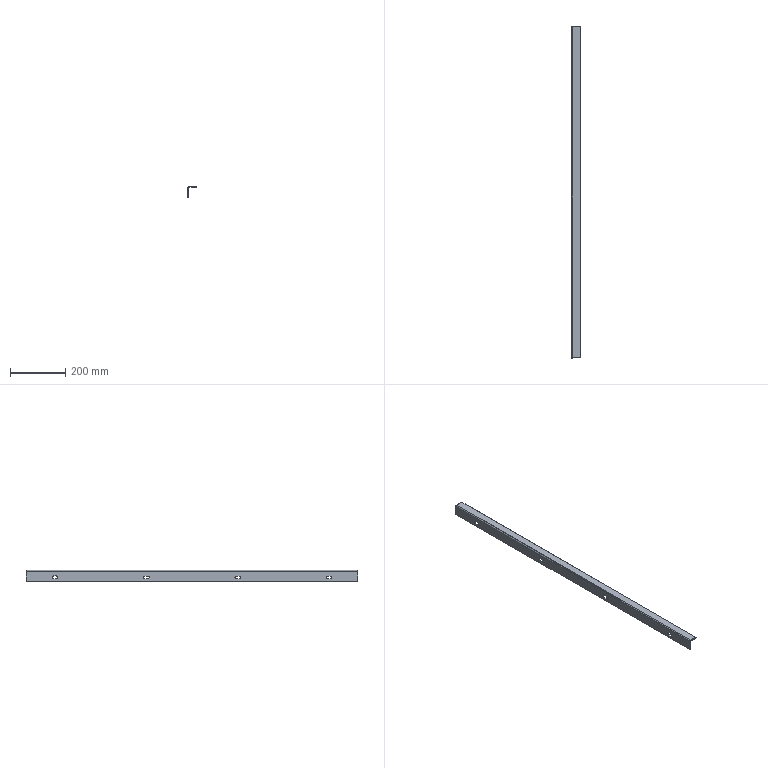Component | SolidWorks | FrontTopCoverAssembly-1_FrontTopCoverStiffener-1 | 1 solid | 38 faces | volume 158496 mm3 | plane 24 | cylinder 14 | commonest cylinder face diameters 10 x12 8 x1 4 x1 | material Plain Carbon Steel